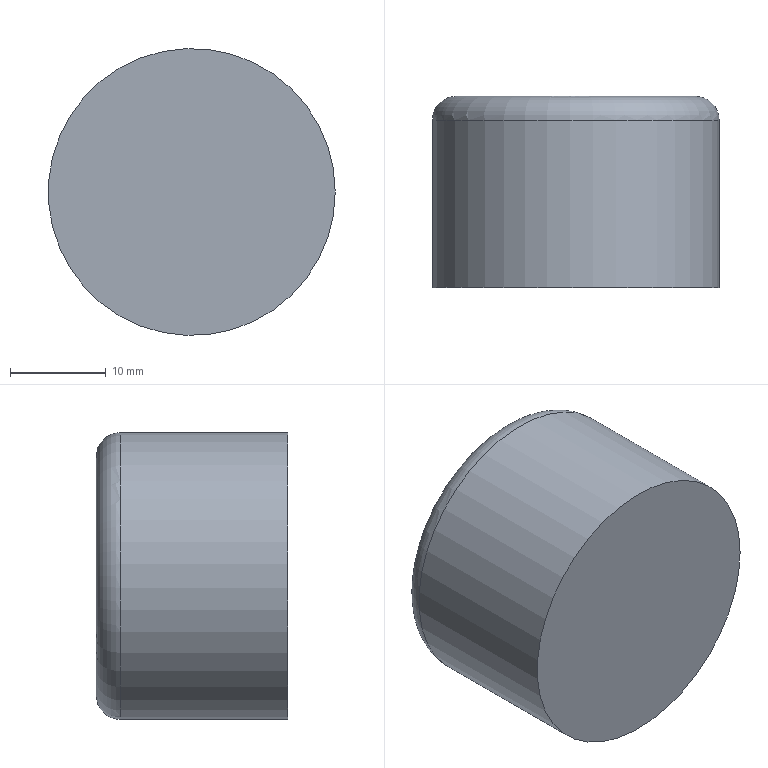Component | NX | BUTTON | 1 solid | 4 faces | box 30 x 20 x 30 mm | volume 14015 mm3 | plane 2 | cylinder 1 | torus 1 | commonest cylinder face diameters 30 x1
STEP:
#1=CARTESIAN_POINT('',(0.,0.,0.));
#2=DIRECTION('',(0.,0.,1.));
#3=DIRECTION('',(1.,0.,0.));
#4=AXIS2_PLACEMENT_3D('',#1,#2,#3);
#5=CARTESIAN_POINT('',(12.5,70.,-322.5));
#6=VERTEX_POINT('',#5);
#7=CARTESIAN_POINT('',(-0.,70.,-322.5));
#8=DIRECTION('',(0.,1.,0.));
#9=DIRECTION('',(1.,0.,0.));
#10=AXIS2_PLACEMENT_3D('',#7,#8,#9);
#11=CIRCLE('',#10,12.5);
#12=CARTESIAN_POINT('',(-0.,70.,-322.5));
#13=DIRECTION('',(0.,1.,0.));
#14=DIRECTION('',(1.,0.,0.));
#15=AXIS2_PLACEMENT_3D('',#12,#13,#14);
#16=PLANE('',#15);
#17=CARTESIAN_POINT('',(0.,0.));
#18=DIRECTION('',(1.,0.));
#19=AXIS2_PLACEMENT_2D('',#17,#18);
#20=CIRCLE('',#19,12.5);
#21=(GEOMETRIC_REPRESENTATION_CONTEXT(2)PARAMETRIC_REPRESENTATION_CONTEXT()REPRESENTATION_CONTEXT('',''));
#22=DEFINITIONAL_REPRESENTATION('',(#20),#21);
#23=PCURVE('',#16,#22);
#24=CARTESIAN_POINT('',(-0.,67.5,-322.5));
#25=DIRECTION('',(0.,1.,0.));
#26=DIRECTION('',(1.,0.,0.));
#27=AXIS2_PLACEMENT_3D('',#24,#25,#26);
#28=TOROIDAL_SURFACE('',#27,12.5,2.5);
#29=CARTESIAN_POINT('',(0.,7.854));
#30=DIRECTION('',(1.,0.));
#31=VECTOR('',#30,1.);
#32=LINE('',#29,#31);
#33=(GEOMETRIC_REPRESENTATION_CONTEXT(2)PARAMETRIC_REPRESENTATION_CONTEXT()REPRESENTATION_CONTEXT('',''));
#34=DEFINITIONAL_REPRESENTATION('',(#32),#33);
#35=PCURVE('',#28,#34);
#36=SURFACE_CURVE('',#11,(#23,#35),.PCURVE_S1.);
#37=EDGE_CURVE('',#6,#6,#36,.T.);
#38=ORIENTED_EDGE('',*,*,#37,.T.);
#39=EDGE_LOOP('',(#38));
#40=FACE_BOUND('',#39,.T.);
#41=ADVANCED_FACE('',(#40),#16,.T.);
#42=CARTESIAN_POINT('',(15.,50.,-322.5));
#43=VERTEX_POINT('',#42);
#44=CARTESIAN_POINT('',(-0.,50.,-322.5));
#45=DIRECTION('',(0.,1.,0.));
#46=DIRECTION('',(1.,0.,0.));
#47=AXIS2_PLACEMENT_3D('',#44,#45,#46);
#48=CIRCLE('',#47,15.);
#49=CARTESIAN_POINT('',(-0.,50.,-322.5));
#50=DIRECTION('',(0.,-1.,0.));
#51=DIRECTION('',(-1.,0.,0.));
#52=AXIS2_PLACEMENT_3D('',#49,#50,#51);
#53=PLANE('',#52);
#54=CARTESIAN_POINT('',(-15.,0.));
#55=CARTESIAN_POINT('',(-15.,25.981));
#56=CARTESIAN_POINT('',(7.5,12.99));
#57=CARTESIAN_POINT('',(30.,0.));
#58=CARTESIAN_POINT('',(7.5,-12.99));
#59=CARTESIAN_POINT('',(-15.,-25.981));
#60=CARTESIAN_POINT('',(-15.,0.));
#61=(BOUNDED_CURVE()B_SPLINE_CURVE(2,(#54,#55,#56,#57,#58,#59,#60),.UNSPECIFIED.,.T.,.F.)B_SPLINE_CURVE_WITH_KNOTS((1,2,2,2,2,1),(-2.094,0.,2.094,4.189,6.283,8.378),.UNSPECIFIED.)CURVE()GEOMETRIC_REPRESENTATION_ITEM()RATIONAL_B_SPLINE_CURVE((1.,0.5,1.,0.5,1.,0.5,1.))REPRESENTATION_ITEM(''));
#62=(GEOMETRIC_REPRESENTATION_CONTEXT(2)PARAMETRIC_REPRESENTATION_CONTEXT()REPRESENTATION_CONTEXT('',''));
#63=DEFINITIONAL_REPRESENTATION('',(#61),#62);
#64=PCURVE('',#53,#63);
#65=CARTESIAN_POINT('',(-0.,50.,-322.5));
#66=DIRECTION('',(0.,1.,0.));
#67=DIRECTION('',(1.,0.,0.));
#68=AXIS2_PLACEMENT_3D('',#65,#66,#67);
#69=CYLINDRICAL_SURFACE('',#68,15.);
#70=CARTESIAN_POINT('',(0.,0.));
#71=DIRECTION('',(1.,0.));
#72=VECTOR('',#71,1.);
#73=LINE('',#70,#72);
#74=(GEOMETRIC_REPRESENTATION_CONTEXT(2)PARAMETRIC_REPRESENTATION_CONTEXT()REPRESENTATION_CONTEXT('',''));
#75=DEFINITIONAL_REPRESENTATION('',(#73),#74);
#76=PCURVE('',#69,#75);
#77=SURFACE_CURVE('',#48,(#64,#76),.PCURVE_S1.);
#78=EDGE_CURVE('',#43,#43,#77,.T.);
#79=ORIENTED_EDGE('',*,*,#78,.F.);
#80=EDGE_LOOP('',(#79));
#81=FACE_BOUND('',#80,.T.);
#82=ADVANCED_FACE('',(#81),#53,.T.);
#83=CARTESIAN_POINT('',(15.,67.5,-322.5));
#84=VERTEX_POINT('',#83);
#85=CARTESIAN_POINT('',(-0.,67.5,-322.5));
#86=DIRECTION('',(0.,-1.,0.));
#87=DIRECTION('',(1.,0.,0.));
#88=AXIS2_PLACEMENT_3D('',#85,#86,#87);
#89=CIRCLE('',#88,15.);
#90=CARTESIAN_POINT('',(6.283,17.5));
#91=DIRECTION('',(-1.,0.));
#92=VECTOR('',#91,1.);
#93=LINE('',#90,#92);
#94=(GEOMETRIC_REPRESENTATION_CONTEXT(2)PARAMETRIC_REPRESENTATION_CONTEXT()REPRESENTATION_CONTEXT('',''));
#95=DEFINITIONAL_REPRESENTATION('',(#93),#94);
#96=PCURVE('',#69,#95);
#97=CARTESIAN_POINT('',(6.283,6.283));
#98=DIRECTION('',(-1.,0.));
#99=VECTOR('',#98,1.);
#100=LINE('',#97,#99);
#101=(GEOMETRIC_REPRESENTATION_CONTEXT(2)PARAMETRIC_REPRESENTATION_CONTEXT()REPRESENTATION_CONTEXT('',''));
#102=DEFINITIONAL_REPRESENTATION('',(#100),#101);
#103=PCURVE('',#28,#102);
#104=SURFACE_CURVE('',#89,(#96,#103),.PCURVE_S1.);
#105=EDGE_CURVE('',#84,#84,#104,.T.);
#106=ORIENTED_EDGE('',*,*,#105,.T.);
#107=CARTESIAN_POINT('',(15.,50.,-322.5));
#108=CARTESIAN_POINT('',(15.,67.5,-322.5));
#109=B_SPLINE_CURVE_WITH_KNOTS('',1,(#107,#108),.UNSPECIFIED.,.F.,.F.,(2,2),(0.,17.5),.PIECEWISE_BEZIER_KNOTS.);
#110=CARTESIAN_POINT('',(0.,0.));
#111=DIRECTION('',(0.,1.));
#112=VECTOR('',#111,1.);
#113=LINE('',#110,#112);
#114=(GEOMETRIC_REPRESENTATION_CONTEXT(2)PARAMETRIC_REPRESENTATION_CONTEXT()REPRESENTATION_CONTEXT('',''));
#115=DEFINITIONAL_REPRESENTATION('',(#113),#114);
#116=PCURVE('',#69,#115);
#117=CARTESIAN_POINT('',(6.283,0.));
#118=DIRECTION('',(0.,1.));
#119=VECTOR('',#118,1.);
#120=LINE('',#117,#119);
#121=(GEOMETRIC_REPRESENTATION_CONTEXT(2)PARAMETRIC_REPRESENTATION_CONTEXT()REPRESENTATION_CONTEXT('',''));
#122=DEFINITIONAL_REPRESENTATION('',(#120),#121);
#123=PCURVE('',#69,#122);
#124=SEAM_CURVE('',#109,(#116,#123),.PCURVE_S1.);
#125=EDGE_CURVE('',#43,#84,#124,.T.);
#126=ORIENTED_EDGE('',*,*,#125,.F.);
#127=ORIENTED_EDGE('',*,*,#78,.T.);
#128=ORIENTED_EDGE('',*,*,#125,.T.);
#129=EDGE_LOOP('',(#106,#126,#127,#128));
#130=FACE_BOUND('',#129,.T.);
#131=ADVANCED_FACE('',(#130),#69,.T.);
#132=ORIENTED_EDGE('',*,*,#37,.F.);
#133=CARTESIAN_POINT('',(15.,67.5,-322.5));
#134=CARTESIAN_POINT('',(15.,68.168,-322.5));
#135=CARTESIAN_POINT('',(14.787,68.819,-322.5));
#136=CARTESIAN_POINT('',(14.38,69.38,-322.5));
#137=CARTESIAN_POINT('',(13.819,69.787,-322.5));
#138=CARTESIAN_POINT('',(13.168,70.,-322.5));
#139=CARTESIAN_POINT('',(12.5,70.,-322.5));
#140=(BOUNDED_CURVE()B_SPLINE_CURVE(6,(#133,#134,#135,#136,#137,#138,#139),.UNSPECIFIED.,.F.,.F.)B_SPLINE_CURVE_WITH_KNOTS((7,7),(0.,1.571),.PIECEWISE_BEZIER_KNOTS.)CURVE()GEOMETRIC_REPRESENTATION_ITEM()RATIONAL_B_SPLINE_CURVE((1.031,1.01,0.9979,0.994,0.9979,1.01,1.031))REPRESENTATION_ITEM(''));
#141=CARTESIAN_POINT('',(0.,6.283));
#142=DIRECTION('',(0.,1.));
#143=VECTOR('',#142,1.);
#144=LINE('',#141,#143);
#145=(GEOMETRIC_REPRESENTATION_CONTEXT(2)PARAMETRIC_REPRESENTATION_CONTEXT()REPRESENTATION_CONTEXT('',''));
#146=DEFINITIONAL_REPRESENTATION('',(#144),#145);
#147=PCURVE('',#28,#146);
#148=CARTESIAN_POINT('',(6.283,6.283));
#149=DIRECTION('',(0.,1.));
#150=VECTOR('',#149,1.);
#151=LINE('',#148,#150);
#152=(GEOMETRIC_REPRESENTATION_CONTEXT(2)PARAMETRIC_REPRESENTATION_CONTEXT()REPRESENTATION_CONTEXT('',''));
#153=DEFINITIONAL_REPRESENTATION('',(#151),#152);
#154=PCURVE('',#28,#153);
#155=SEAM_CURVE('',#140,(#147,#154),.PCURVE_S1.);
#156=EDGE_CURVE('',#84,#6,#155,.T.);
#157=ORIENTED_EDGE('',*,*,#156,.F.);
#158=ORIENTED_EDGE('',*,*,#105,.F.);
#159=ORIENTED_EDGE('',*,*,#156,.T.);
#160=EDGE_LOOP('',(#132,#157,#158,#159));
#161=FACE_BOUND('',#160,.T.);
#162=ADVANCED_FACE('',(#161),#28,.T.);
#163=CLOSED_SHELL('',(#41,#82,#131,#162));
#164=MANIFOLD_SOLID_BREP('',#163);
#165=(LENGTH_UNIT()NAMED_UNIT(*)SI_UNIT(.MILLI.,.METRE.));
#166=UNCERTAINTY_MEASURE_WITH_UNIT(LENGTH_MEASURE(0.00001),#165,'','');
#167=(NAMED_UNIT(*)PLANE_ANGLE_UNIT()SI_UNIT($,.RADIAN.));
#168=(NAMED_UNIT(*)SI_UNIT($,.STERADIAN.)SOLID_ANGLE_UNIT());
#169=(GEOMETRIC_REPRESENTATION_CONTEXT(3)GLOBAL_UNCERTAINTY_ASSIGNED_CONTEXT((#166))GLOBAL_UNIT_ASSIGNED_CONTEXT((#165,#167,#168))REPRESENTATION_CONTEXT('',''));
#170=ADVANCED_BREP_SHAPE_REPRESENTATION('',(#4,#164),#169);